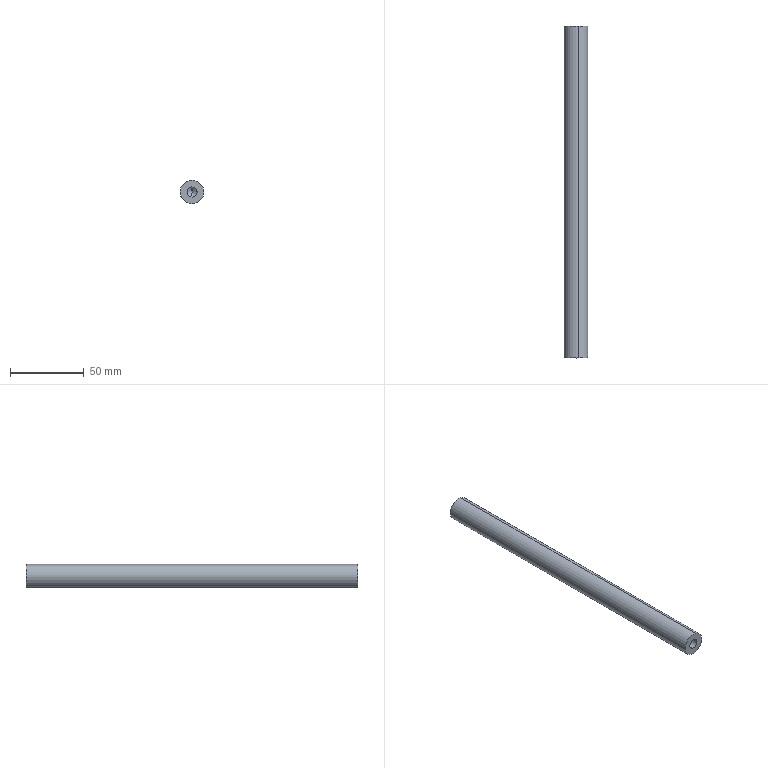Component | SolidWorks | GuideRod-3 | 1 solid | 8 faces | box 16.03 x 225 x 16 mm | volume 44406 mm3 | cylinder 4 | cone 2 | plane 2 | commonest cylinder face diameters 6.8 x2 16 x2 | material AISI 304
build123d program:
from build123d import *

# Parameters (mm, degrees)
SKETCH1_R             = 8
BOSS_EXTRUDE1_DEPTH   = 112.5
M8_TAPPED_HOLE1_D     = 6.8
M8_TAPPED_HOLE1_DEPTH = 22.25
M8_TAPPED_HOLE1_TIP   = 2.043


with BuildPart() as part:
    # Sketch1 → Boss-Extrude1 (new, symmetric)
    with BuildSketch(Plane.XY):
        Circle(SKETCH1_R)
    extrude(amount=BOSS_EXTRUDE1_DEPTH, both=True)

    # M8 Tapped Hole1
    with Locations(Plane(origin=(0, 0, -112.5), x_dir=(-1, 0, 0), z_dir=(0, 0, -1))):
        with Locations((0, 0)):
            Hole(M8_TAPPED_HOLE1_D / 2, depth=M8_TAPPED_HOLE1_DEPTH)
            with Locations((0, 0, -(M8_TAPPED_HOLE1_DEPTH + M8_TAPPED_HOLE1_TIP / 2))):  # 118° drill point
                Cone(0, M8_TAPPED_HOLE1_D / 2, M8_TAPPED_HOLE1_TIP, mode=Mode.SUBTRACT)


solid = part.part

# Placed as in the assembly
solid = solid.moved(Location((1612.13, 4048.956, 1079.241), (-90, -0.008895, -0.003657)))
STEP:
#1=COLOUR_RGB('',0.7922,0.8196,0.9333);
#2=FILL_AREA_STYLE_COLOUR('',#1);
#3=FILL_AREA_STYLE('',(#2));
#4=SURFACE_STYLE_FILL_AREA(#3);
#5=SURFACE_SIDE_STYLE('',(#4));
#6=SURFACE_STYLE_USAGE(.BOTH.,#5);
#7=PRESENTATION_STYLE_ASSIGNMENT((#6));
#8=CARTESIAN_POINT('',(63.439,155.855,42.36));
#9=VERTEX_POINT('',#8);
#10=CARTESIAN_POINT('',(63.501,155.855,42.62));
#11=VERTEX_POINT('',#10);
#12=CARTESIAN_POINT('',(63.47,155.855,42.49));
#13=DIRECTION('',(0.0001552,-1.,-0.));
#14=DIRECTION('',(0.2336,0.00003626,0.9723));
#15=AXIS2_PLACEMENT_3D('',#12,#13,#14);
#16=CIRCLE('',#15,0.1339);
#17=EDGE_CURVE('',#9,#11,#16,.T.);
#18=ORIENTED_EDGE('',*,*,#17,.F.);
#19=CARTESIAN_POINT('',(63.439,154.979,42.36));
#20=VERTEX_POINT('',#19);
#21=CARTESIAN_POINT('',(63.439,154.979,42.36));
#22=DIRECTION('',(0.0001552,-1.,-0.));
#23=VECTOR('',#22,39.37);
#24=LINE('',#21,#23);
#25=EDGE_CURVE('',#9,#20,#24,.T.);
#26=ORIENTED_EDGE('',*,*,#25,.T.);
#27=CARTESIAN_POINT('',(63.502,154.979,42.62));
#28=VERTEX_POINT('',#27);
#29=CARTESIAN_POINT('',(63.47,154.979,42.49));
#30=DIRECTION('',(0.0001552,-1.,-0.));
#31=DIRECTION('',(0.2336,0.00003626,0.9723));
#32=AXIS2_PLACEMENT_3D('',#29,#30,#31);
#33=CIRCLE('',#32,0.1339);
#34=EDGE_CURVE('',#20,#28,#33,.T.);
#35=ORIENTED_EDGE('',*,*,#34,.T.);
#36=CARTESIAN_POINT('',(63.502,154.979,42.62));
#37=DIRECTION('',(0.0001552,-1.,-0.));
#38=VECTOR('',#37,39.37);
#39=LINE('',#36,#38);
#40=EDGE_CURVE('',#11,#28,#39,.T.);
#41=ORIENTED_EDGE('',*,*,#40,.F.);
#42=EDGE_LOOP('',(#18,#26,#35,#41));
#43=FACE_OUTER_BOUND('',#42,.T.);
#44=CARTESIAN_POINT('',(63.47,154.979,42.49));
#45=DIRECTION('',(0.0001552,-1.,-0.));
#46=DIRECTION('',(0.2336,0.00003626,0.9723));
#47=AXIS2_PLACEMENT_3D('',#44,#45,#46);
#48=CYLINDRICAL_SURFACE('',#47,0.1339);
#49=ADVANCED_FACE('',(#43),#48,.F.);
#50=CARTESIAN_POINT('',(63.47,155.935,42.49));
#51=VERTEX_POINT('',#50);
#52=CARTESIAN_POINT('',(63.501,155.855,42.62));
#53=DIRECTION('',(0.2003,-0.515,0.8335));
#54=VECTOR('',#53,39.37);
#55=LINE('',#52,#54);
#56=EDGE_CURVE('',#51,#11,#55,.T.);
#57=ORIENTED_EDGE('',*,*,#56,.F.);
#58=CARTESIAN_POINT('',(63.439,155.855,42.36));
#59=DIRECTION('',(-0.2001,-0.5151,-0.8335));
#60=VECTOR('',#59,39.37);
#61=LINE('',#58,#60);
#62=EDGE_CURVE('',#51,#9,#61,.T.);
#63=ORIENTED_EDGE('',*,*,#62,.T.);
#64=ORIENTED_EDGE('',*,*,#17,.T.);
#65=EDGE_LOOP('',(#57,#63,#64));
#66=FACE_OUTER_BOUND('',#65,.T.);
#67=CARTESIAN_POINT('',(63.47,155.855,42.49));
#68=DIRECTION('',(0.0001552,-1.,-0.));
#69=DIRECTION('',(0.2336,0.00003626,0.9723));
#70=AXIS2_PLACEMENT_3D('',#67,#68,#69);
#71=CONICAL_SURFACE('',#70,0.1339,1.03);
#72=ADVANCED_FACE('',(#66),#71,.F.);
#73=CARTESIAN_POINT('',(63.395,163.837,42.184));
#74=VERTEX_POINT('',#73);
#75=CARTESIAN_POINT('',(63.543,163.837,42.796));
#76=VERTEX_POINT('',#75);
#77=CARTESIAN_POINT('',(63.469,163.837,42.49));
#78=DIRECTION('',(-0.0001552,1.,0.));
#79=DIRECTION('',(-0.2336,-0.00003626,-0.9723));
#80=AXIS2_PLACEMENT_3D('',#77,#78,#79);
#81=CIRCLE('',#80,0.315);
#82=EDGE_CURVE('',#74,#76,#81,.T.);
#83=ORIENTED_EDGE('',*,*,#82,.F.);
#84=CARTESIAN_POINT('',(63.397,154.979,42.184));
#85=VERTEX_POINT('',#84);
#86=CARTESIAN_POINT('',(63.395,163.837,42.184));
#87=DIRECTION('',(0.0001552,-1.,-0.));
#88=VECTOR('',#87,39.37);
#89=LINE('',#86,#88);
#90=EDGE_CURVE('',#74,#85,#89,.T.);
#91=ORIENTED_EDGE('',*,*,#90,.T.);
#92=CARTESIAN_POINT('',(63.544,154.979,42.796));
#93=VERTEX_POINT('',#92);
#94=CARTESIAN_POINT('',(63.47,154.979,42.49));
#95=DIRECTION('',(-0.0001552,1.,0.));
#96=DIRECTION('',(-0.2336,-0.00003626,-0.9723));
#97=AXIS2_PLACEMENT_3D('',#94,#95,#96);
#98=CIRCLE('',#97,0.315);
#99=EDGE_CURVE('',#85,#93,#98,.T.);
#100=ORIENTED_EDGE('',*,*,#99,.T.);
#101=CARTESIAN_POINT('',(63.543,163.837,42.796));
#102=DIRECTION('',(0.0001552,-1.,-0.));
#103=VECTOR('',#102,39.37);
#104=LINE('',#101,#103);
#105=EDGE_CURVE('',#76,#93,#104,.T.);
#106=ORIENTED_EDGE('',*,*,#105,.F.);
#107=EDGE_LOOP('',(#83,#91,#100,#106));
#108=FACE_OUTER_BOUND('',#107,.T.);
#109=CARTESIAN_POINT('',(63.469,163.837,42.49));
#110=DIRECTION('',(0.0001552,-1.,-0.));
#111=DIRECTION('',(0.2336,0.00003626,0.9723));
#112=AXIS2_PLACEMENT_3D('',#109,#110,#111);
#113=CYLINDRICAL_SURFACE('',#112,0.315);
#114=ADVANCED_FACE('',(#108),#113,.T.);
#115=ORIENTED_EDGE('',*,*,#90,.F.);
#116=CARTESIAN_POINT('',(63.469,163.837,42.49));
#117=DIRECTION('',(-0.0001552,1.,0.));
#118=DIRECTION('',(-0.2336,-0.00003626,-0.9723));
#119=AXIS2_PLACEMENT_3D('',#116,#117,#118);
#120=CIRCLE('',#119,0.315);
#121=EDGE_CURVE('',#76,#74,#120,.T.);
#122=ORIENTED_EDGE('',*,*,#121,.F.);
#123=ORIENTED_EDGE('',*,*,#105,.T.);
#124=CARTESIAN_POINT('',(63.47,154.979,42.49));
#125=DIRECTION('',(-0.0001552,1.,0.));
#126=DIRECTION('',(-0.2336,-0.00003626,-0.9723));
#127=AXIS2_PLACEMENT_3D('',#124,#125,#126);
#128=CIRCLE('',#127,0.315);
#129=EDGE_CURVE('',#93,#85,#128,.T.);
#130=ORIENTED_EDGE('',*,*,#129,.T.);
#131=EDGE_LOOP('',(#115,#122,#123,#130));
#132=FACE_OUTER_BOUND('',#131,.T.);
#133=CARTESIAN_POINT('',(63.469,163.837,42.49));
#134=DIRECTION('',(0.0001552,-1.,-0.));
#135=DIRECTION('',(0.2336,0.00003626,0.9723));
#136=AXIS2_PLACEMENT_3D('',#133,#134,#135);
#137=CYLINDRICAL_SURFACE('',#136,0.315);
#138=ADVANCED_FACE('',(#132),#137,.T.);
#139=ORIENTED_EDGE('',*,*,#121,.T.);
#140=ORIENTED_EDGE('',*,*,#82,.T.);
#141=EDGE_LOOP('',(#139,#140));
#142=FACE_OUTER_BOUND('',#141,.T.);
#143=CARTESIAN_POINT('',(63.469,163.837,42.49));
#144=DIRECTION('',(-0.0001552,1.,0.));
#145=DIRECTION('',(-0.2336,-0.00003626,-0.9723));
#146=AXIS2_PLACEMENT_3D('',#143,#144,#145);
#147=PLANE('',#146);
#148=ADVANCED_FACE('',(#142),#147,.T.);
#149=CARTESIAN_POINT('',(63.47,154.979,42.49));
#150=DIRECTION('',(0.0001552,-1.,-0.));
#151=DIRECTION('',(0.2336,0.00003626,0.9723));
#152=AXIS2_PLACEMENT_3D('',#149,#150,#151);
#153=CIRCLE('',#152,0.1339);
#154=EDGE_CURVE('',#28,#20,#153,.T.);
#155=ORIENTED_EDGE('',*,*,#154,.F.);
#156=ORIENTED_EDGE('',*,*,#34,.F.);
#157=EDGE_LOOP('',(#155,#156));
#158=FACE_BOUND('',#157,.T.);
#159=ORIENTED_EDGE('',*,*,#129,.F.);
#160=ORIENTED_EDGE('',*,*,#99,.F.);
#161=EDGE_LOOP('',(#159,#160));
#162=FACE_OUTER_BOUND('',#161,.T.);
#163=CARTESIAN_POINT('',(63.47,154.979,42.49));
#164=DIRECTION('',(-0.0001552,1.,0.));
#165=DIRECTION('',(-0.2336,-0.00003626,-0.9723));
#166=AXIS2_PLACEMENT_3D('',#163,#164,#165);
#167=PLANE('',#166);
#168=ADVANCED_FACE('',(#158,#162),#167,.F.);
#169=ORIENTED_EDGE('',*,*,#62,.F.);
#170=ORIENTED_EDGE('',*,*,#56,.T.);
#171=CARTESIAN_POINT('',(63.47,155.855,42.49));
#172=DIRECTION('',(0.0001552,-1.,-0.));
#173=DIRECTION('',(0.2336,0.00003626,0.9723));
#174=AXIS2_PLACEMENT_3D('',#171,#172,#173);
#175=CIRCLE('',#174,0.1339);
#176=EDGE_CURVE('',#11,#9,#175,.T.);
#177=ORIENTED_EDGE('',*,*,#176,.T.);
#178=EDGE_LOOP('',(#169,#170,#177));
#179=FACE_OUTER_BOUND('',#178,.T.);
#180=CARTESIAN_POINT('',(63.47,155.855,42.49));
#181=DIRECTION('',(0.0001552,-1.,-0.));
#182=DIRECTION('',(0.2336,0.00003626,0.9723));
#183=AXIS2_PLACEMENT_3D('',#180,#181,#182);
#184=CONICAL_SURFACE('',#183,0.1339,1.03);
#185=ADVANCED_FACE('',(#179),#184,.F.);
#186=ORIENTED_EDGE('',*,*,#25,.F.);
#187=ORIENTED_EDGE('',*,*,#176,.F.);
#188=ORIENTED_EDGE('',*,*,#40,.T.);
#189=ORIENTED_EDGE('',*,*,#154,.T.);
#190=EDGE_LOOP('',(#186,#187,#188,#189));
#191=FACE_OUTER_BOUND('',#190,.T.);
#192=CARTESIAN_POINT('',(63.47,154.979,42.49));
#193=DIRECTION('',(0.0001552,-1.,-0.));
#194=DIRECTION('',(0.2336,0.00003626,0.9723));
#195=AXIS2_PLACEMENT_3D('',#192,#193,#194);
#196=CYLINDRICAL_SURFACE('',#195,0.1339);
#197=ADVANCED_FACE('',(#191),#196,.F.);
#198=CLOSED_SHELL('',(#49,#72,#114,#138,#148,#168,#185,#197));
#199=MANIFOLD_SOLID_BREP('',#198);
#200=STYLED_ITEM('',(#7),#199);
#201=(LENGTH_UNIT()NAMED_UNIT(*)SI_UNIT($,.METRE.));
#202=LENGTH_MEASURE_WITH_UNIT(LENGTH_MEASURE(0.0254),#201);
#203=DIMENSIONAL_EXPONENTS(1.,0.,0.,0.,0.,0.,0.);
#204=(CONVERSION_BASED_UNIT('',#202)LENGTH_UNIT()NAMED_UNIT(#203));
#205=UNCERTAINTY_MEASURE_WITH_UNIT(LENGTH_MEASURE(0.00001),#204,'','');
#206=(NAMED_UNIT(*)PLANE_ANGLE_UNIT()SI_UNIT($,.RADIAN.));
#207=(NAMED_UNIT(*)SI_UNIT($,.STERADIAN.)SOLID_ANGLE_UNIT());
#208=(GEOMETRIC_REPRESENTATION_CONTEXT(3)GLOBAL_UNCERTAINTY_ASSIGNED_CONTEXT((#205))GLOBAL_UNIT_ASSIGNED_CONTEXT((#204,#206,#207))REPRESENTATION_CONTEXT('',''));
#209=MECHANICAL_DESIGN_GEOMETRIC_PRESENTATION_REPRESENTATION('',(#200),#208);
#210=CARTESIAN_POINT('',(0.,0.,0.));
#211=DIRECTION('',(0.,0.,1.));
#212=DIRECTION('',(1.,0.,0.));
#213=AXIS2_PLACEMENT_3D('',#210,#211,#212);
#214=(LENGTH_UNIT()NAMED_UNIT(*)SI_UNIT($,.METRE.));
#215=LENGTH_MEASURE_WITH_UNIT(LENGTH_MEASURE(0.0254),#214);
#216=DIMENSIONAL_EXPONENTS(1.,0.,0.,0.,0.,0.,0.);
#217=(CONVERSION_BASED_UNIT('',#215)LENGTH_UNIT()NAMED_UNIT(#216));
#218=UNCERTAINTY_MEASURE_WITH_UNIT(LENGTH_MEASURE(0.00001),#217,'','');
#219=(NAMED_UNIT(*)PLANE_ANGLE_UNIT()SI_UNIT($,.RADIAN.));
#220=(NAMED_UNIT(*)SI_UNIT($,.STERADIAN.)SOLID_ANGLE_UNIT());
#221=(GEOMETRIC_REPRESENTATION_CONTEXT(3)GLOBAL_UNCERTAINTY_ASSIGNED_CONTEXT((#218))GLOBAL_UNIT_ASSIGNED_CONTEXT((#217,#219,#220))REPRESENTATION_CONTEXT('',''));
#222=ADVANCED_BREP_SHAPE_REPRESENTATION('',(#199,#213),#221);
#223=PRESENTATION_LAYER_ASSIGNMENT('','',(#200));